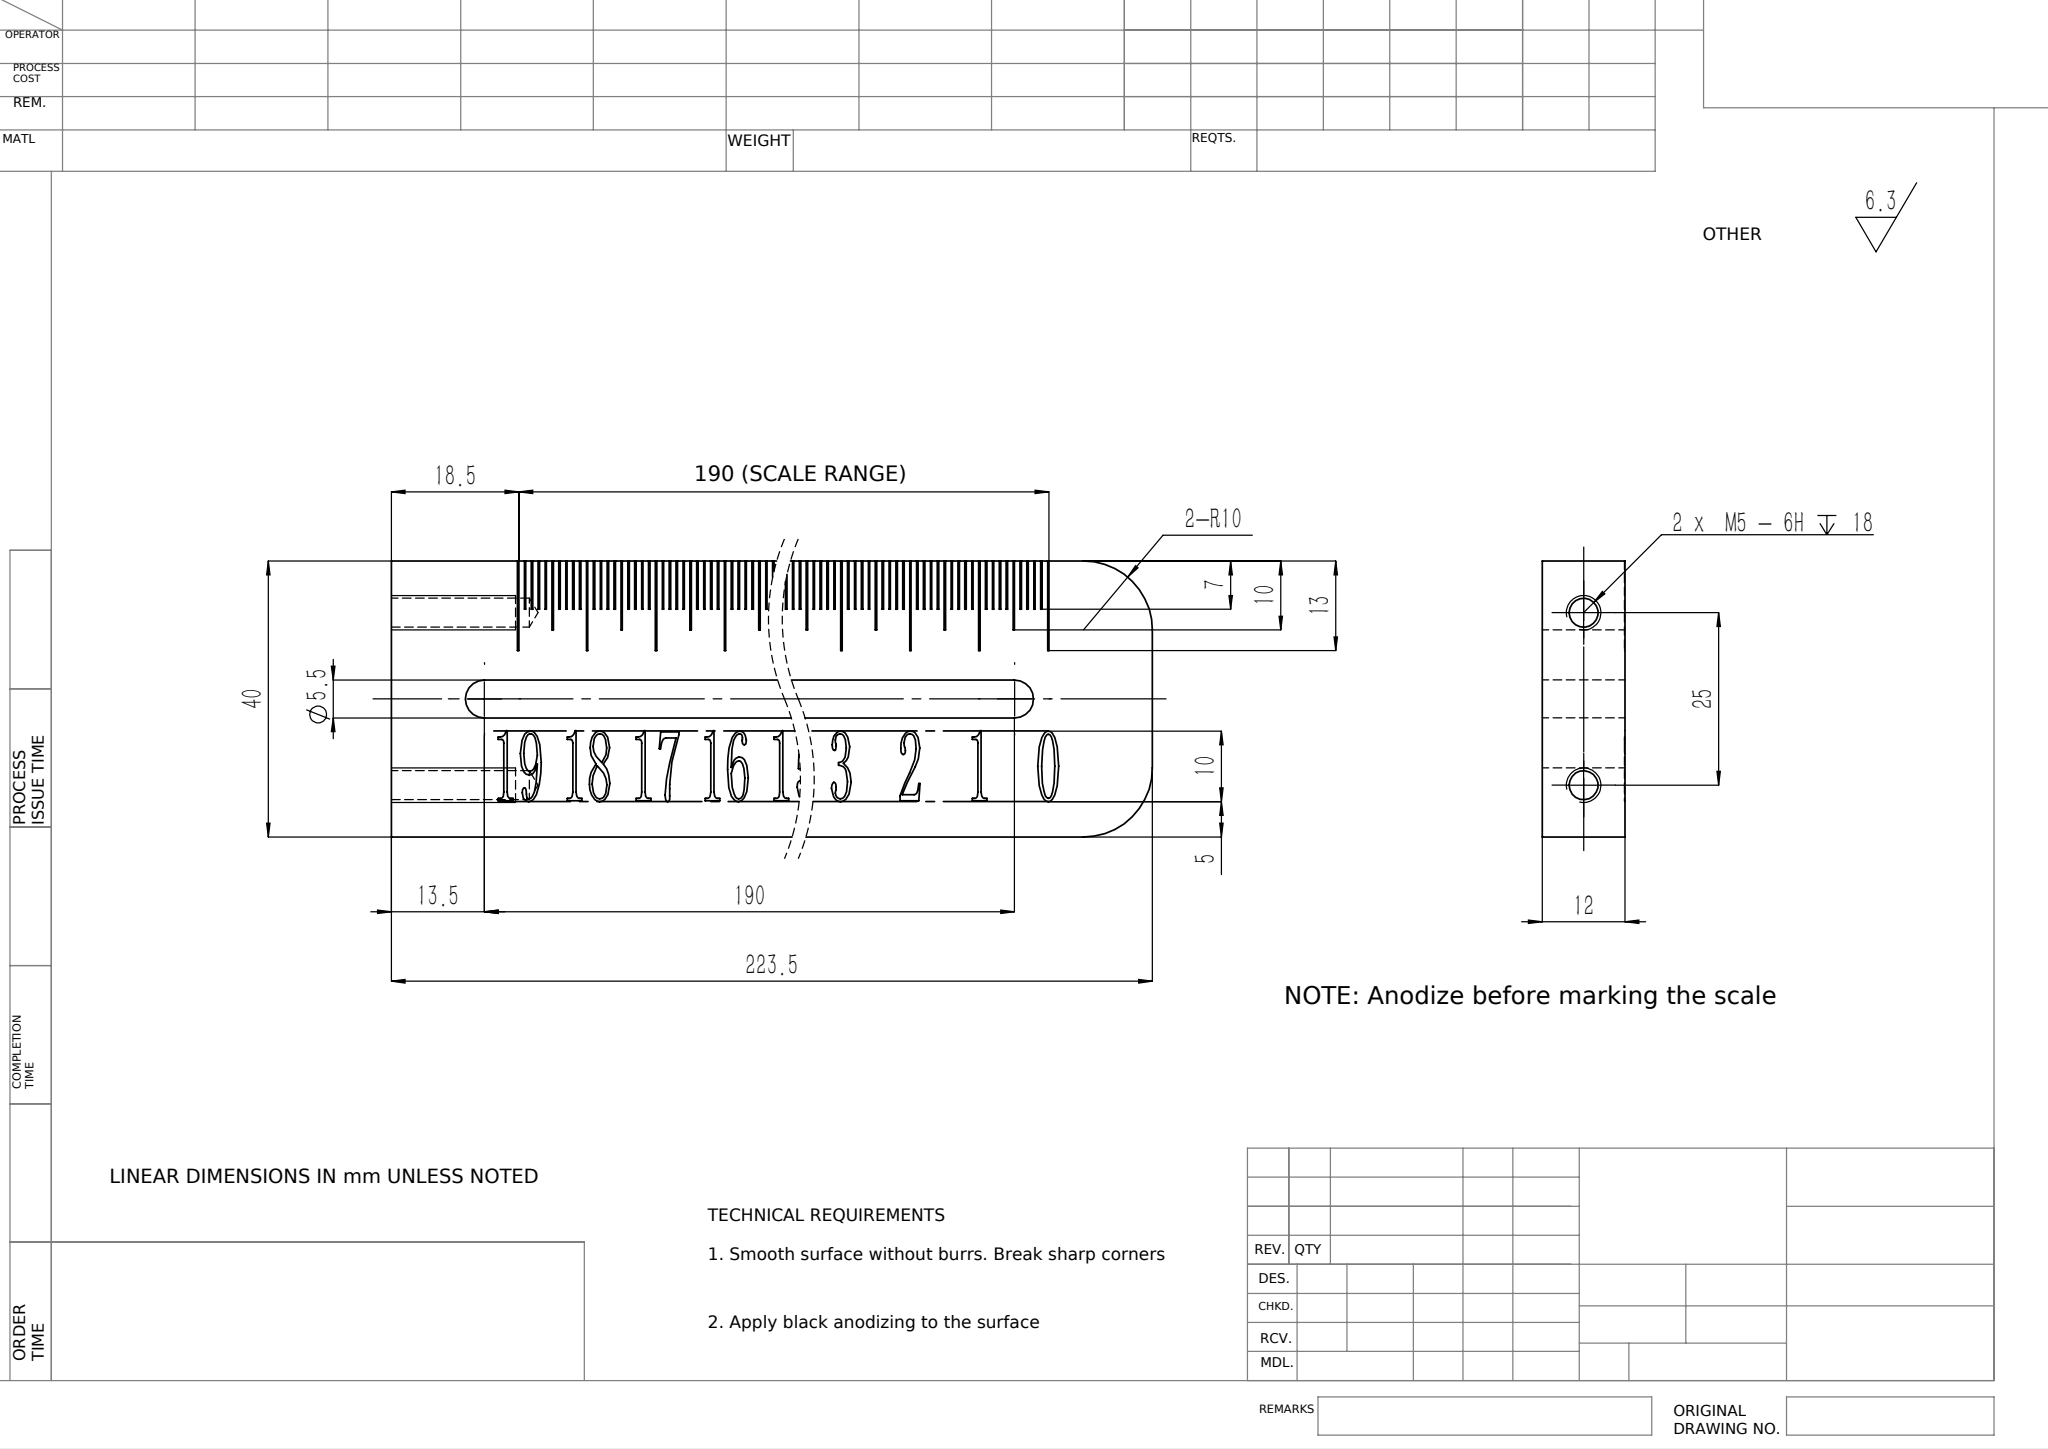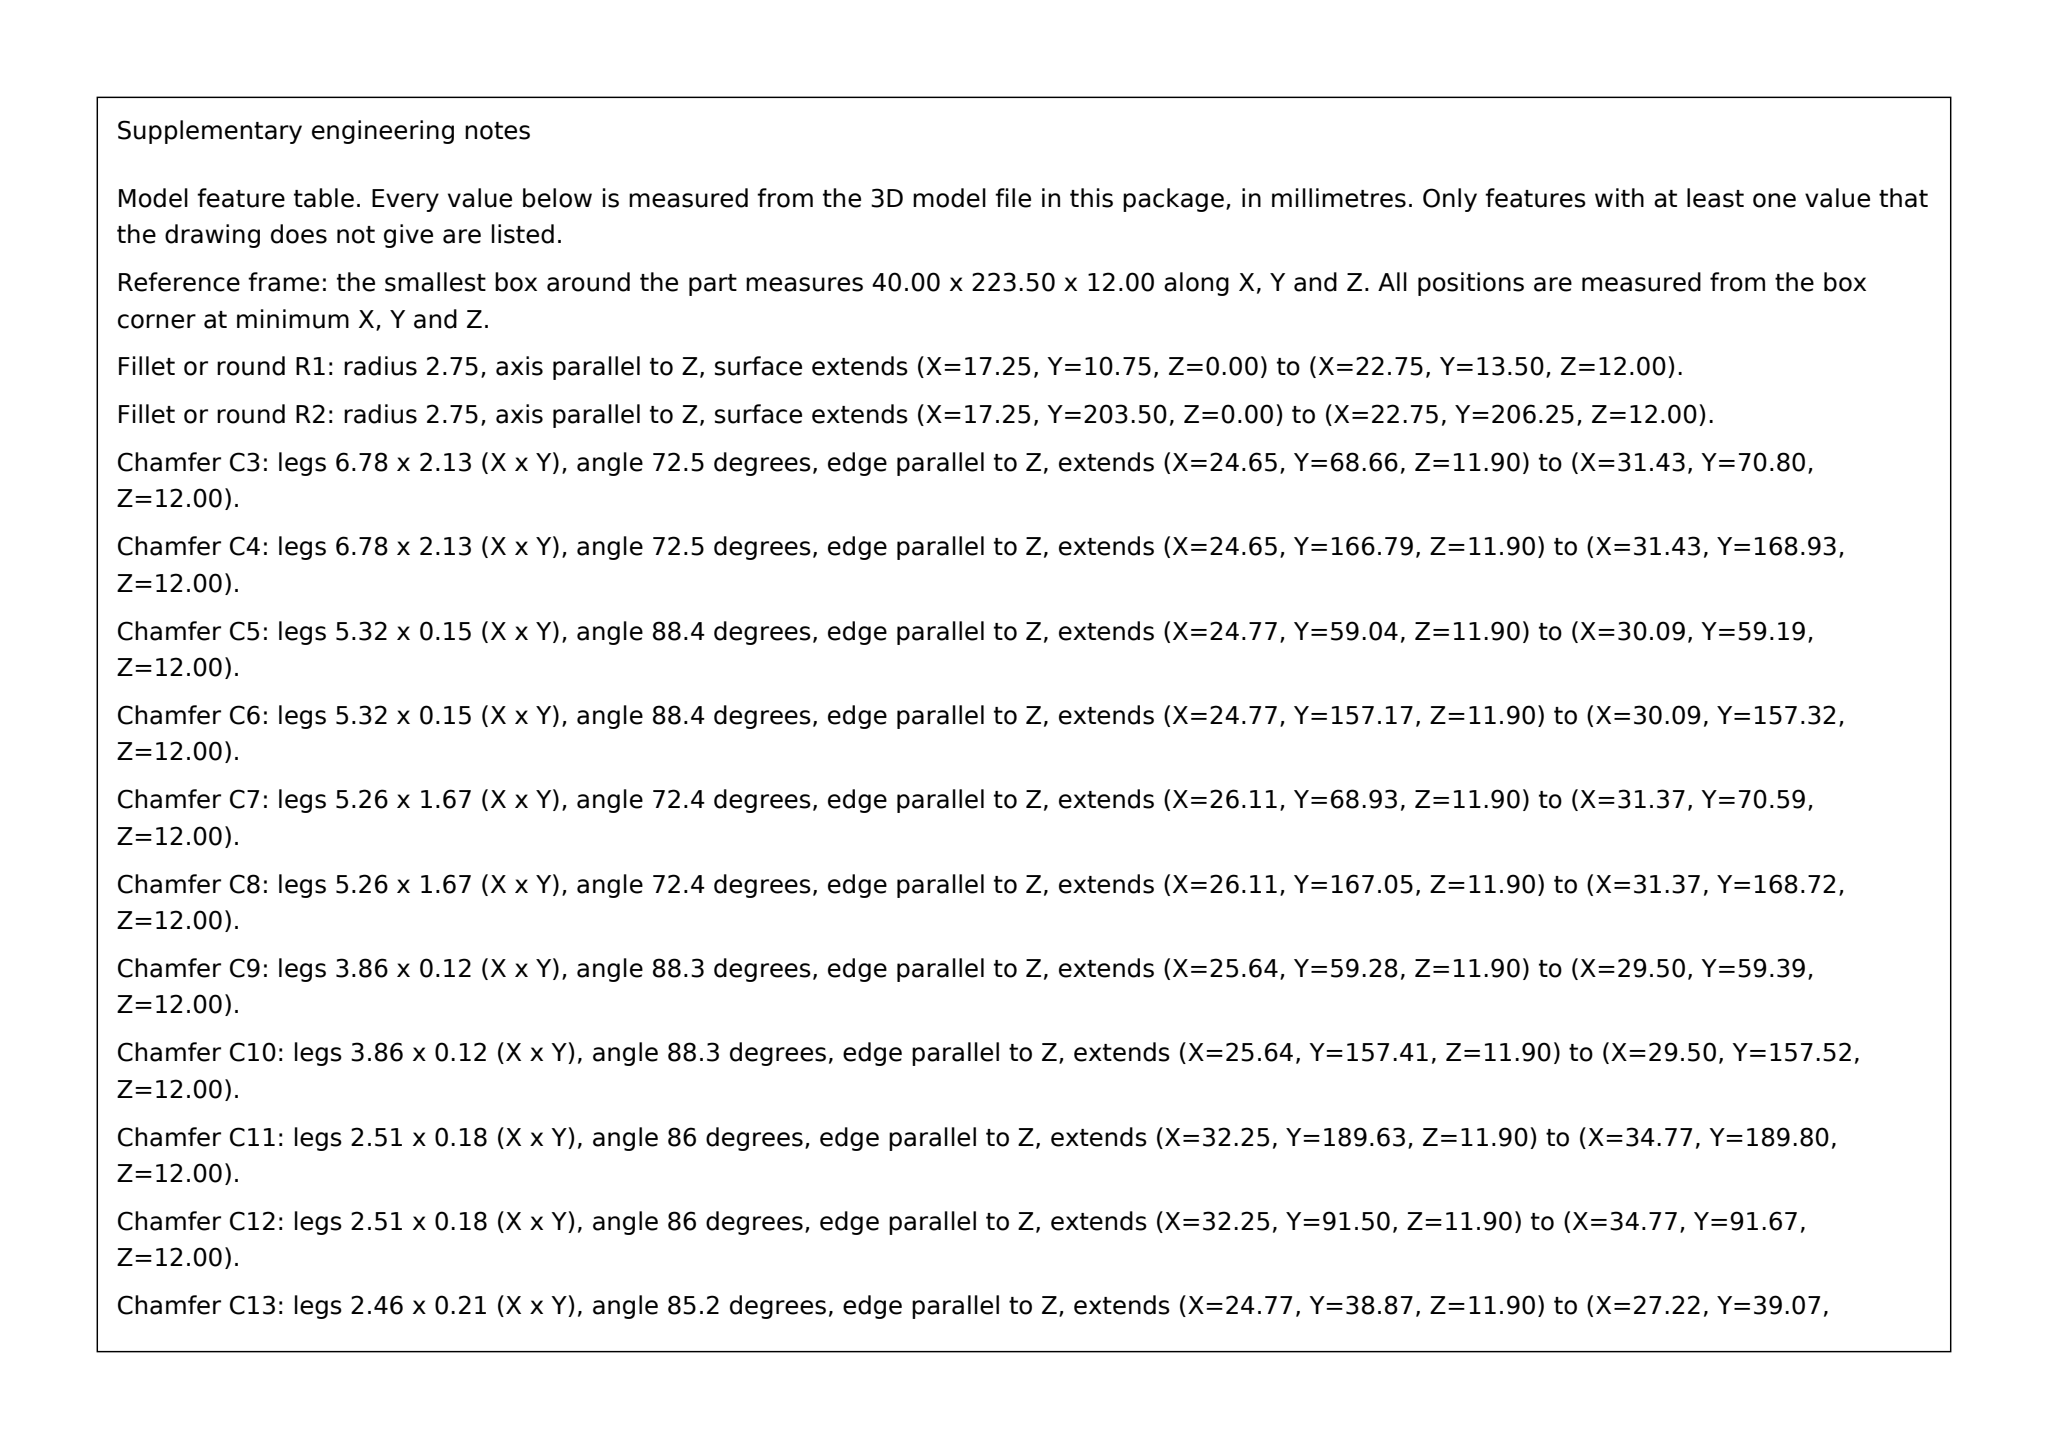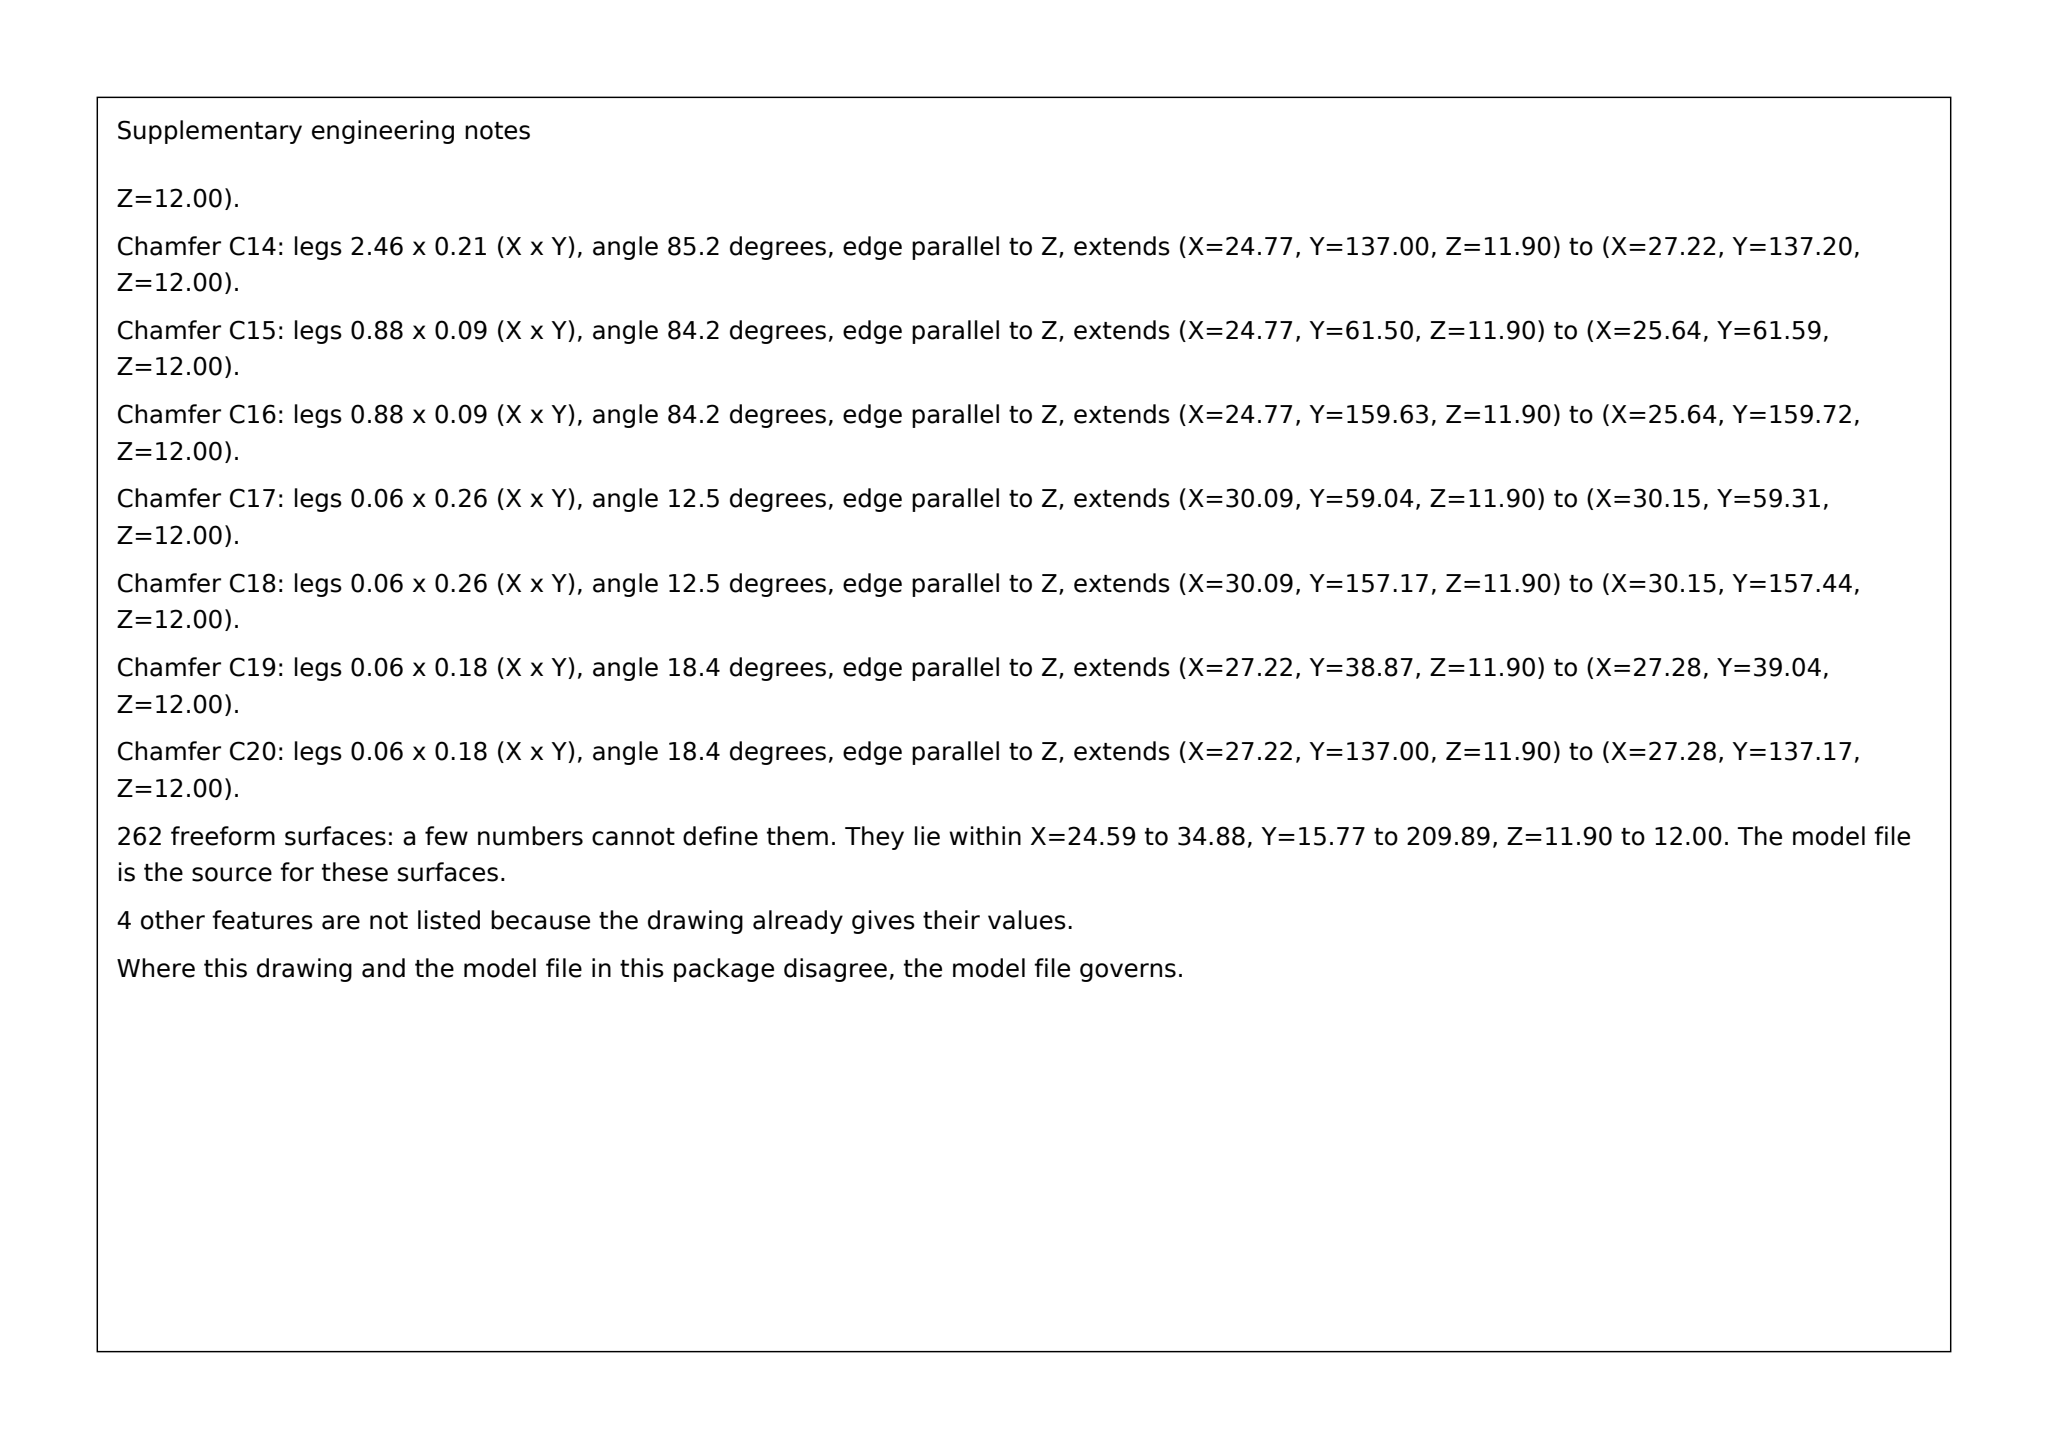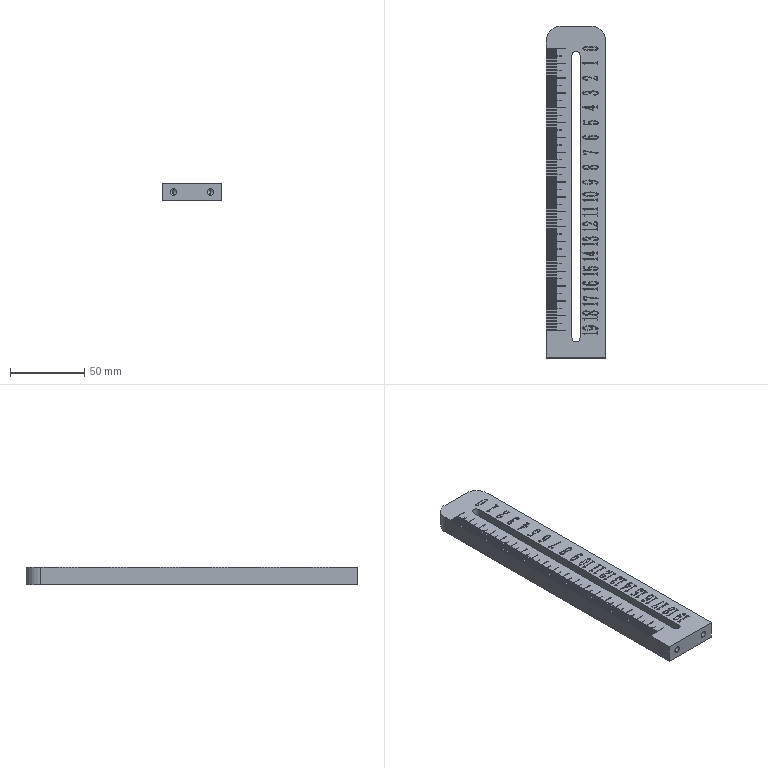Part | SolidWorks | mm | 1 solid | 1296 faces | box 40 x 223.5 x 12 mm | volume 93321 mm3 | plane 1022 | spline 262 | cylinder 8 | cone 4 | commonest cylinder face diameters 4.2 x4 20 x2 5.5 x2